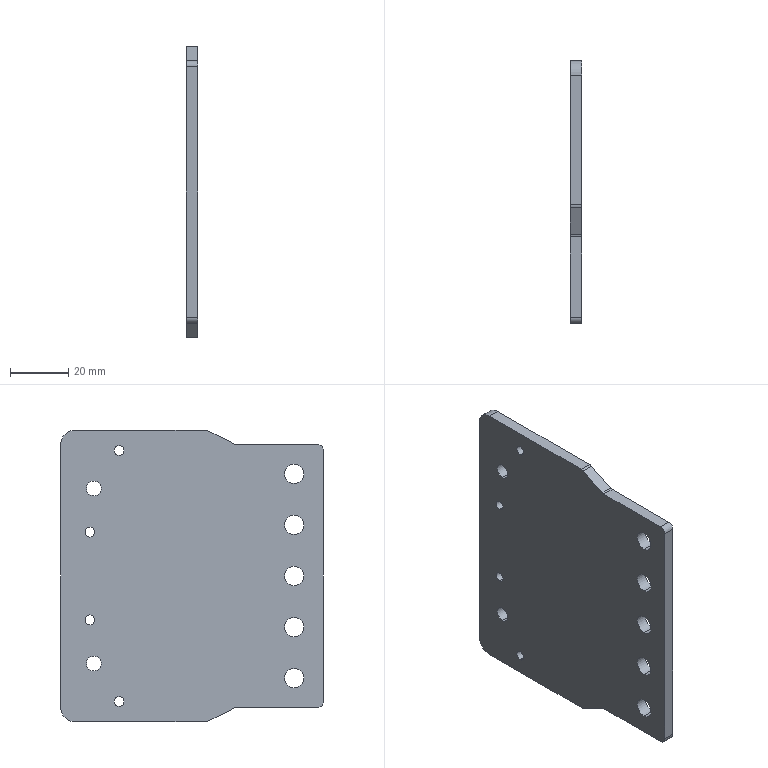Component | SolidWorks | QX1-14-BJV-BracketB-1 | 1 solid | 40 faces | box 4 x 90 x 100 mm | volume 33566 mm3 | cylinder 30 | plane 10 | commonest cylinder face diameters 6.6 x10 3.3 x8 4 x6 5.1 x4 10 x2 | material Q235
build123d program:
from build123d import *

# Parameters (mm, degrees)
BOSS_EXTRUDE1_DEPTH  = 4
M5_CLEARANCE_HOLE1_D = 5.1
FILLET2_R            = 5
FILLET3_R            = 2
M6_CLEARANCE_HOLE1_D = 6.6
M4_TAPPED_HOLE1_D    = 3.3


with BuildPart() as part:
    # Sketch1 → Boss-Extrude1 (new body)
    with BuildSketch(Plane.XY):
        Polygon((-45, 90), (45, 90), (45, 60), (50, 50), (50, 0), (-50, 0), (-50, 50), (-45, 60), align=None)
    extrude(amount=BOSS_EXTRUDE1_DEPTH)

    # M5 Clearance Hole1 (through all)
    with Locations(Plane.XY.offset(4)):
        with Locations((-30, 11.383), (30, 11.383)):
            Hole(M5_CLEARANCE_HOLE1_D / 2)

    # Fillet2
    fillet2_edges = [part.edges().sort_by_distance(p)[0] for p in [
        (50, 0, 2),
        (-50, 0, 2),
    ]]
    fillet(fillet2_edges, radius=FILLET2_R)

    # Fillet3
    fillet3_edges = [part.edges().sort_by_distance(p)[0] for p in [
        (-45, 60, 2),
        (-45, 90, 2),
        (45, 90, 2),
        (45, 60, 2),
        (50, 50, 2),
        (-50, 50, 2),
    ]]
    fillet(fillet3_edges, radius=FILLET3_R)

    # M6 Clearance Hole1 (through all)
    with Locations(Plane(origin=(0, 0, 0), x_dir=(-1, 0, 0), z_dir=(0, 0, -1))):
        with Locations((35, 80), (0, 80), (-35, 80), (-17.5, 80), (17.5, 80)):
            Hole(M6_CLEARANCE_HOLE1_D / 2)

    # M4 Tapped Hole1 (through all)
    with Locations(Plane(origin=(0, 0, 0), x_dir=(-1, 0, 0), z_dir=(0, 0, -1))):
        with Locations((43, 20), (15, 10), (-15, 10), (-43, 20)):
            Hole(M4_TAPPED_HOLE1_D / 2)


solid = part.part

# Placed as in the assembly
solid = solid.moved(Location((-23, 102, 0), (180, 90, 0)))